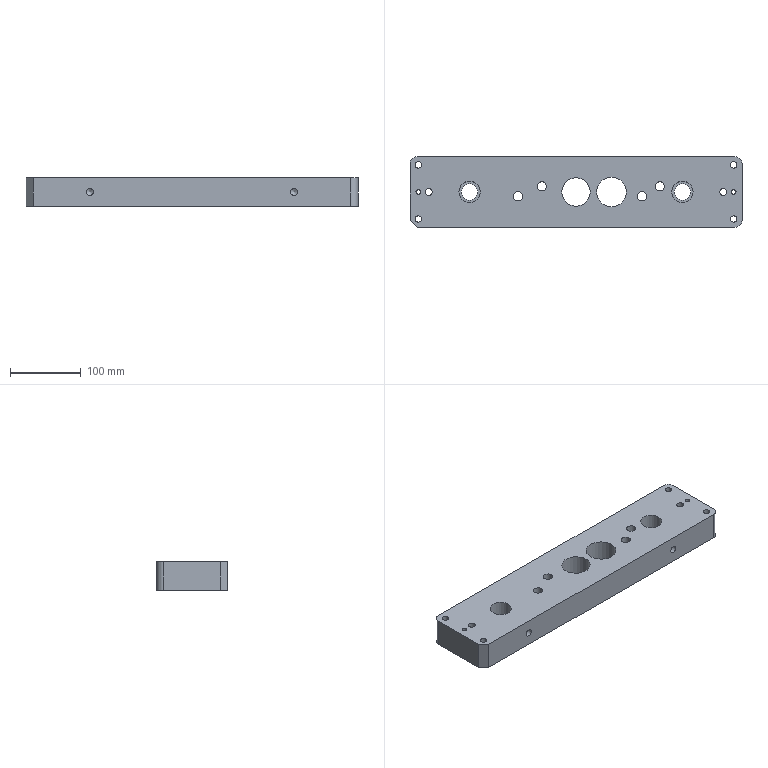CAM job | NX | mm | 3-axis | 3 set-ups | 41 operations | part box 468 x 100 x 40
set-up 1
1. Volume Based 2.5D Milling | Mill Mill5 D100R0.8 | VOLUME_BASED_2.5D_MILLING_1 | path 639 mm | 0.7601 min
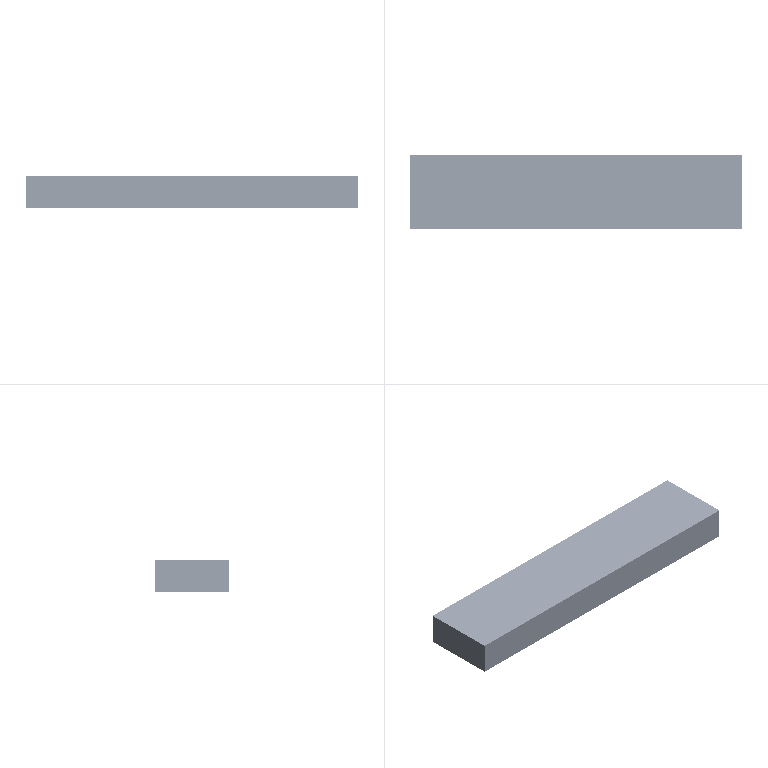2. Point to Point | Mill MillChamfer DXZ-D10A90 | POINT_TO_POINT_2 | path 861.559 mm | 1.349 min
3. Point to Point | Drill DrillStandard ZT-D10.0 | POINT_TO_POINT_3 | path 1083.886 mm | 7.353 min
4. Point to Point | Drill DrillStandard ZT-D9.0 | POINT_TO_POINT_4 | path 1195.419 mm | 5.517 min
5. Point to Point | Drill DrillStandard ZT-D6.6 | POINT_TO_POINT_5 | path 663.432 mm | 1.837 min
6. Point to Point | Drill DrillStandard ZT-D3.3 | POINT_TO_POINT_6 | path 202.152 mm | 0.6829 min
7. Cylinder Milling | Mill Mill5 LX-D12 | CYLINDER_MILLING_7 | path 3237.099 mm | 3.544 min
8. Cylinder Milling | Mill Mill5 LX-D12 | CYLINDER_MILLING_8 | path 2284.15 mm | 2.382 min
9. Planar Milling | Mill Mill5 LX-D12 | PLANAR_MILLING_9 | path 22883.899 mm | 10.278 min
10. Volume Based 2.5D Milling | Mill Mill5 LX-D12 | VOLUME_BASED_2.5D_MILLING_10 | path 727.695 mm | 0.2356 min
11. Planar Roughing | Mill Mill5 LX-D12 | PLANAR_ROUGHING_11 | path 12658.123 mm | 2.712 min
12. Cylinder Milling | Mill Mill5 LX-D10 | CYLINDER_MILLING_12 | path 2615.744 mm | 2.308 min
13. Cylinder Milling | Mill Mill5 LX-D8 | CYLINDER_MILLING_13 | path 1453.379 mm | 1.165 min
14. Cylinder Milling | Mill Mill5 LX-D8 | CYLINDER_MILLING_14 | path 1305.617 mm | 1.013 min
15. Cylinder Milling | Mill Mill5 LX-D12J | CYLINDER_MILLING_15 | path 2027.929 mm | 3.941 min
16. Cylinder Milling | Mill Mill5 LX-D12J | CYLINDER_MILLING_16 | path 868.584 mm | 1.203 min
17. Planar Milling | Mill Mill5 LX-D12J | PLANAR_MILLING_17 | path 747.031 mm | 0.5265 min
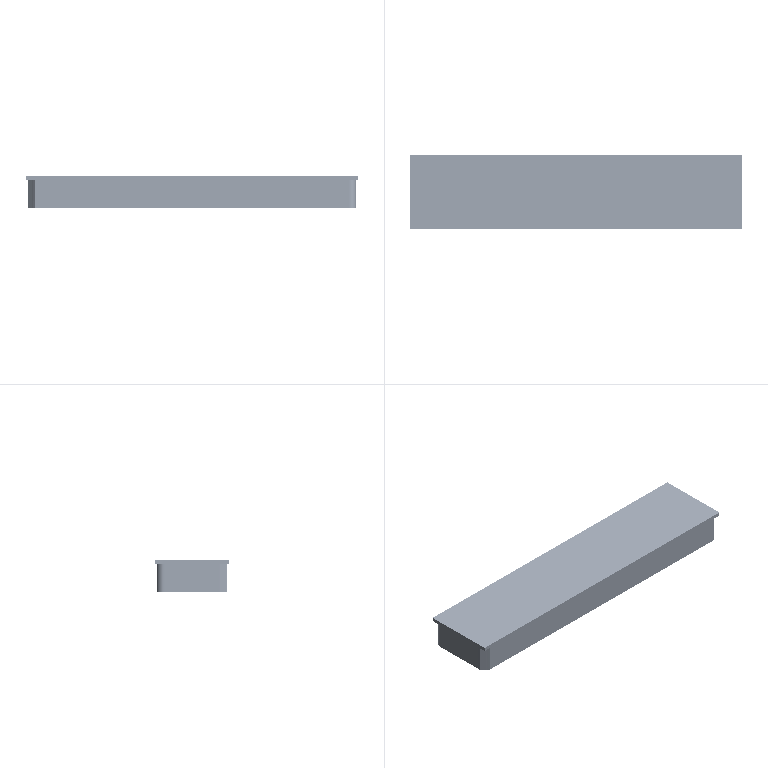18. Volume Based 2.5D Milling | Mill Mill5 LX-D12J | VOLUME_BASED_2.5D_MILLING_18 | path 180.441 mm | 0.1799 min
19. Planar Milling | Mill Mill5 LX-D12J | PLANAR_MILLING_19 | path 2489.741 mm | 2.922 min
20. Cylinder Milling | Mill Mill5 LX-D10J | CYLINDER_MILLING_20 | path 1849.509 mm | 2.615 min
21. Cylinder Milling | Mill Mill5 LX-D8J | CYLINDER_MILLING_21 | path 937.563 mm | 0.9831 min
22. Cylinder Milling | Mill Mill5 LX-D8J | CYLINDER_MILLING_22 | path 863.848 mm | 0.8676 min
23. Volume Based 2.5D Milling | Mill MillChamfer DJ-D10A90 | VOLUME_BASED_2.5D_MILLING_23 | path 200.681 mm | 0.1638 min
24. Planar Milling | Mill MillChamfer DJ-D10A90 | PLANAR_MILLING_24 | path 174.81 mm | 0.1266 min
25. Drilling | Mill MillChamfer DJ-D10A90 | DRILLING_25 | path 225.531 mm | 0.3208 min
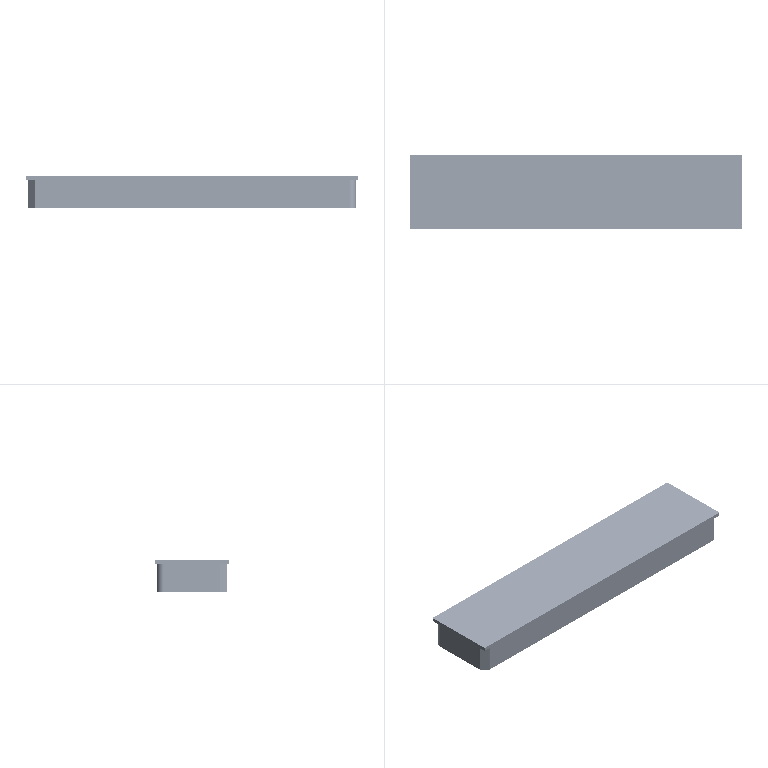26. Planar Text | Mill Mill5 KZ-D0.5R0.25 | PLANAR_TEXT | path 1286.063 mm | 0.378 min
set-up 2
27. Volume Based 2.5D Milling | Mill Mill5 D100R0.8 | VOLUME_BASED_2.5D_MILLING_27 | path 6170.263 mm | 4.022 min
28. Planar Milling | Mill Mill5 LX-D12 | PLANAR_MILLING_28 | path 9333.818 mm | 4.183 min
29. Planar Milling | Mill Mill5 LX-D12 | PLANAR_MILLING_29 | path 5081.361 mm | 2.184 min
30. Cylinder Milling | Mill Mill5 LX-D8 | CYLINDER_MILLING_30 | path 1871.009 mm | 1.866 min
31. Cylinder Milling | Mill Mill5 LX-D6 | CYLINDER_MILLING_31 | path 1307.947 mm | 1.038 min
32. Volume Based 2.5D Milling | Mill Mill5 D100R0.8 | VOLUME_BASED_2.5D_MILLING_32 | path 1249.437 mm | 1.519 min
33. Planar Milling | Mill Mill5 LX-D12J | PLANAR_MILLING_33 | path 804.682 mm | 0.3894 min
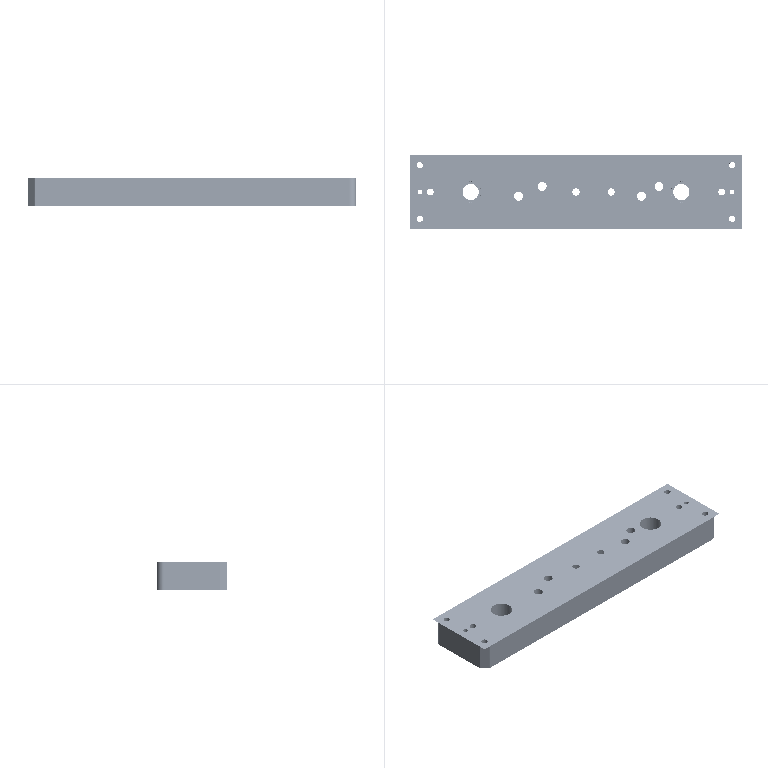34. Planar Milling | Mill Mill5 LX-D12J | PLANAR_MILLING_34 | path 650.482 mm | 0.2191 min
35. Cylinder Milling | Mill Mill5 LX-D6J | CYLINDER_MILLING_35 | path 764.341 mm | 0.6621 min
36. Cylinder Milling | Mill Mill5 LX-D8J | CYLINDER_MILLING_36 | path 1050.744 mm | 1.543 min
37. Fixed-axis Surface Contouring | Mill MillChamfer DJ-D10A90 | FIXED-AXIS_SURFACE_CONTOURING_37 | path 3512.197 mm | 2.615 min
set-up 3
38. Drilling | Mill MillChamfer DXZ-D10A90 | DRILLING_38 | path 372 mm | 0.1697 min
39. Drilling | Drill DrillStandard ZT-D10.3 | DRILLING_39 | path 713.5 mm | 7.026 min
40. Thread Milling | Drill DrillThreadMill M12X1.75-D10_ | THREAD_MILLING_40 | path 1765.868 mm | 2.601 min
41. Thread Milling | Drill DrillThreadMill M12X1.75-D10_ | THREAD_MILLING_41 | path 568.394 mm | 0.4627 min